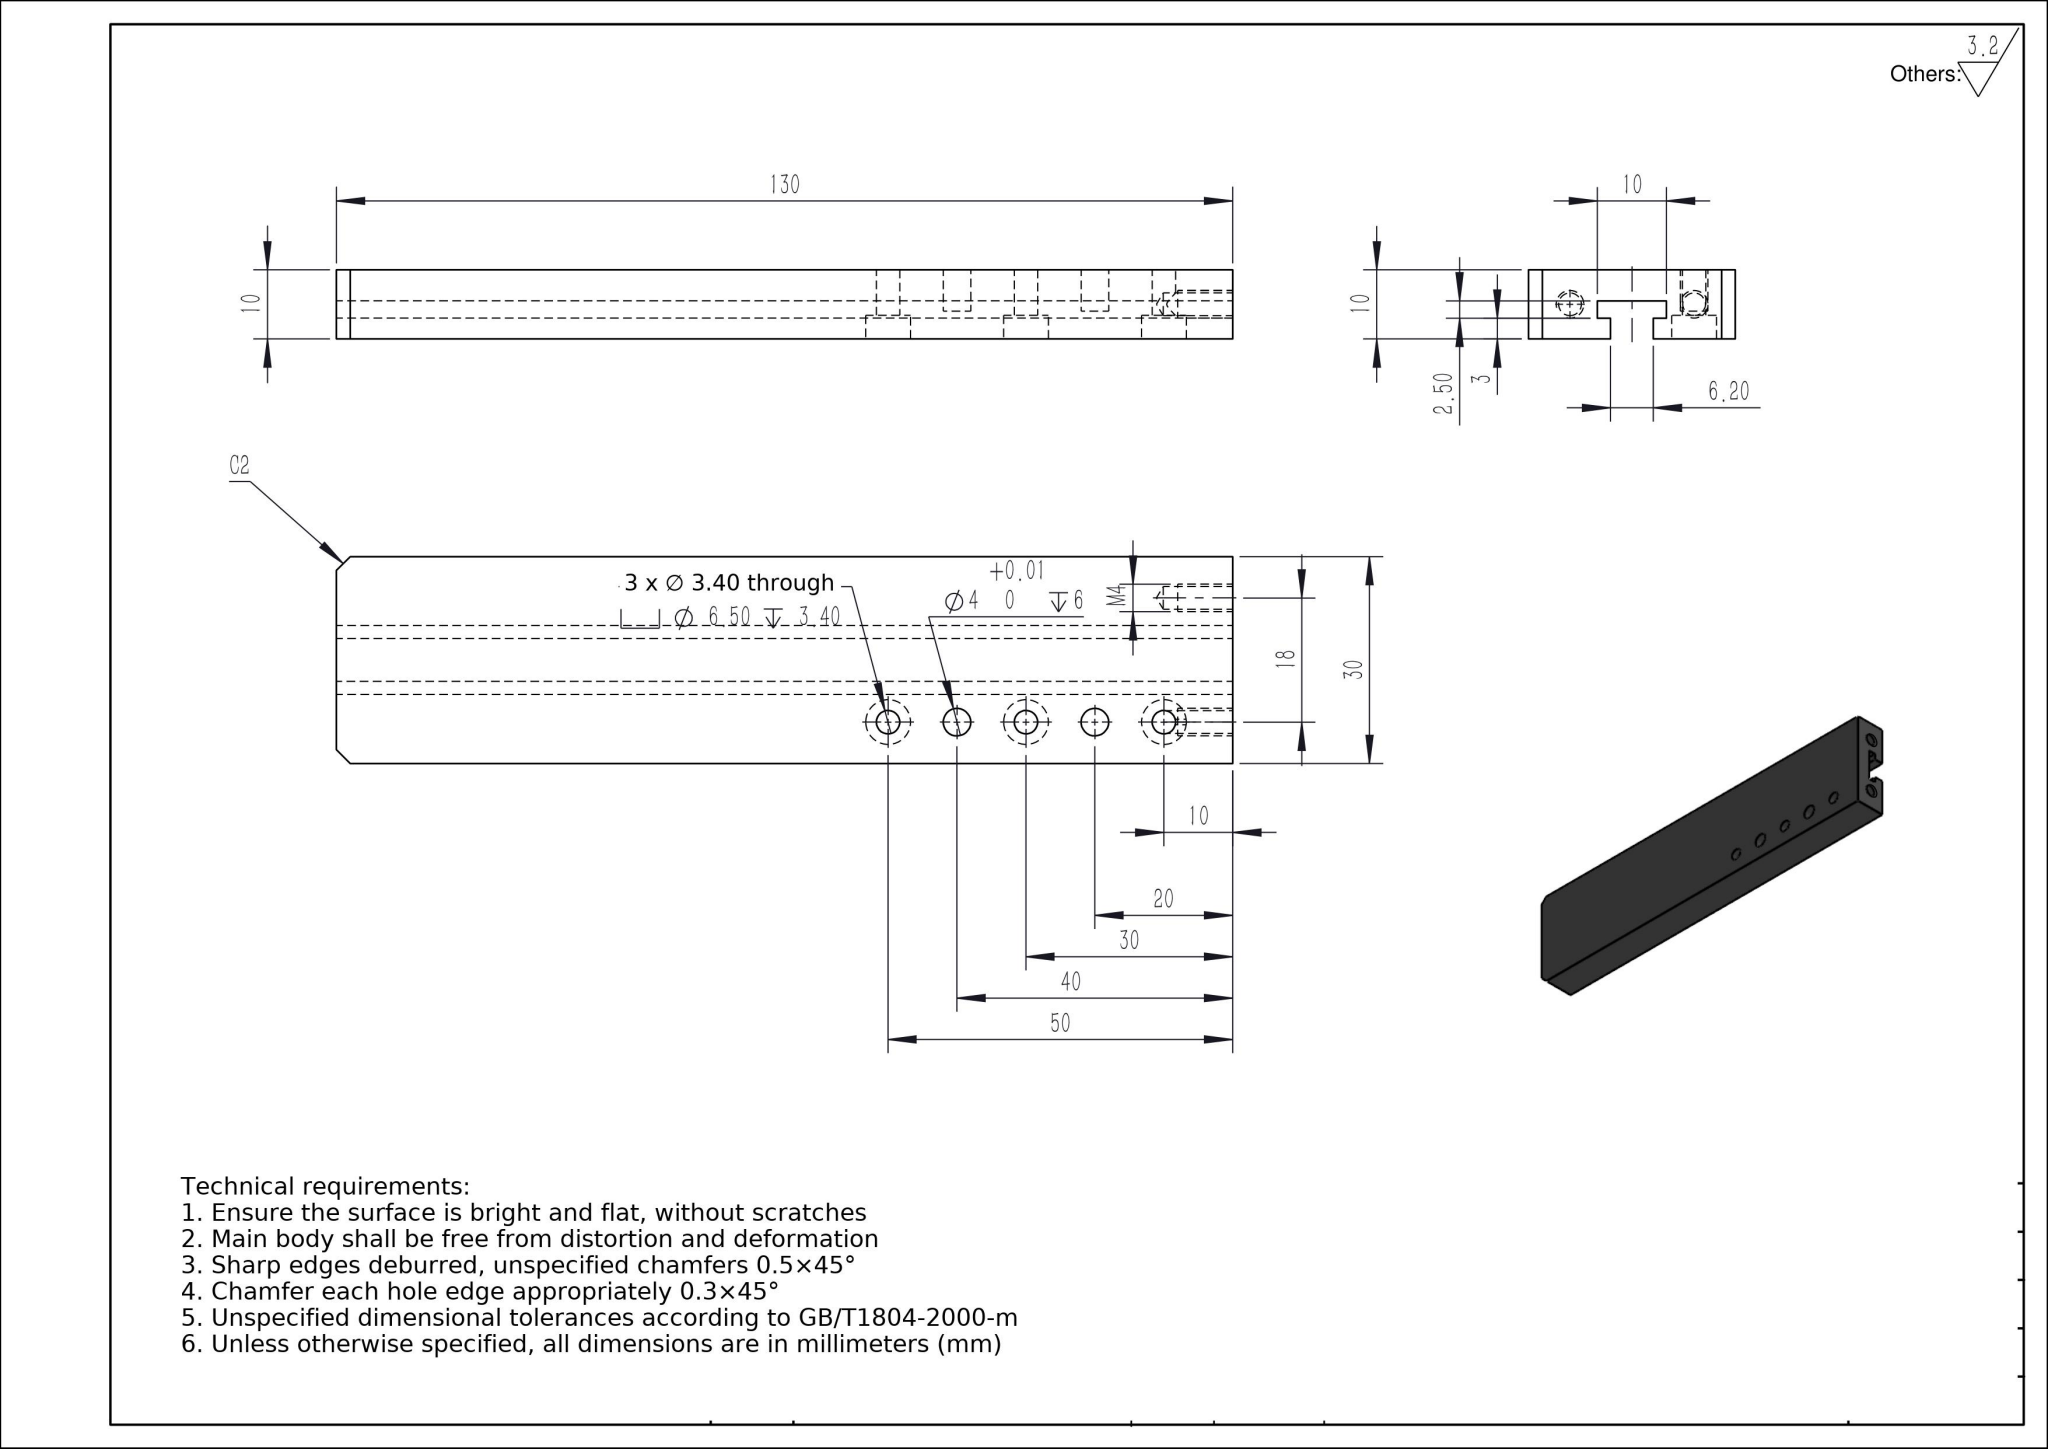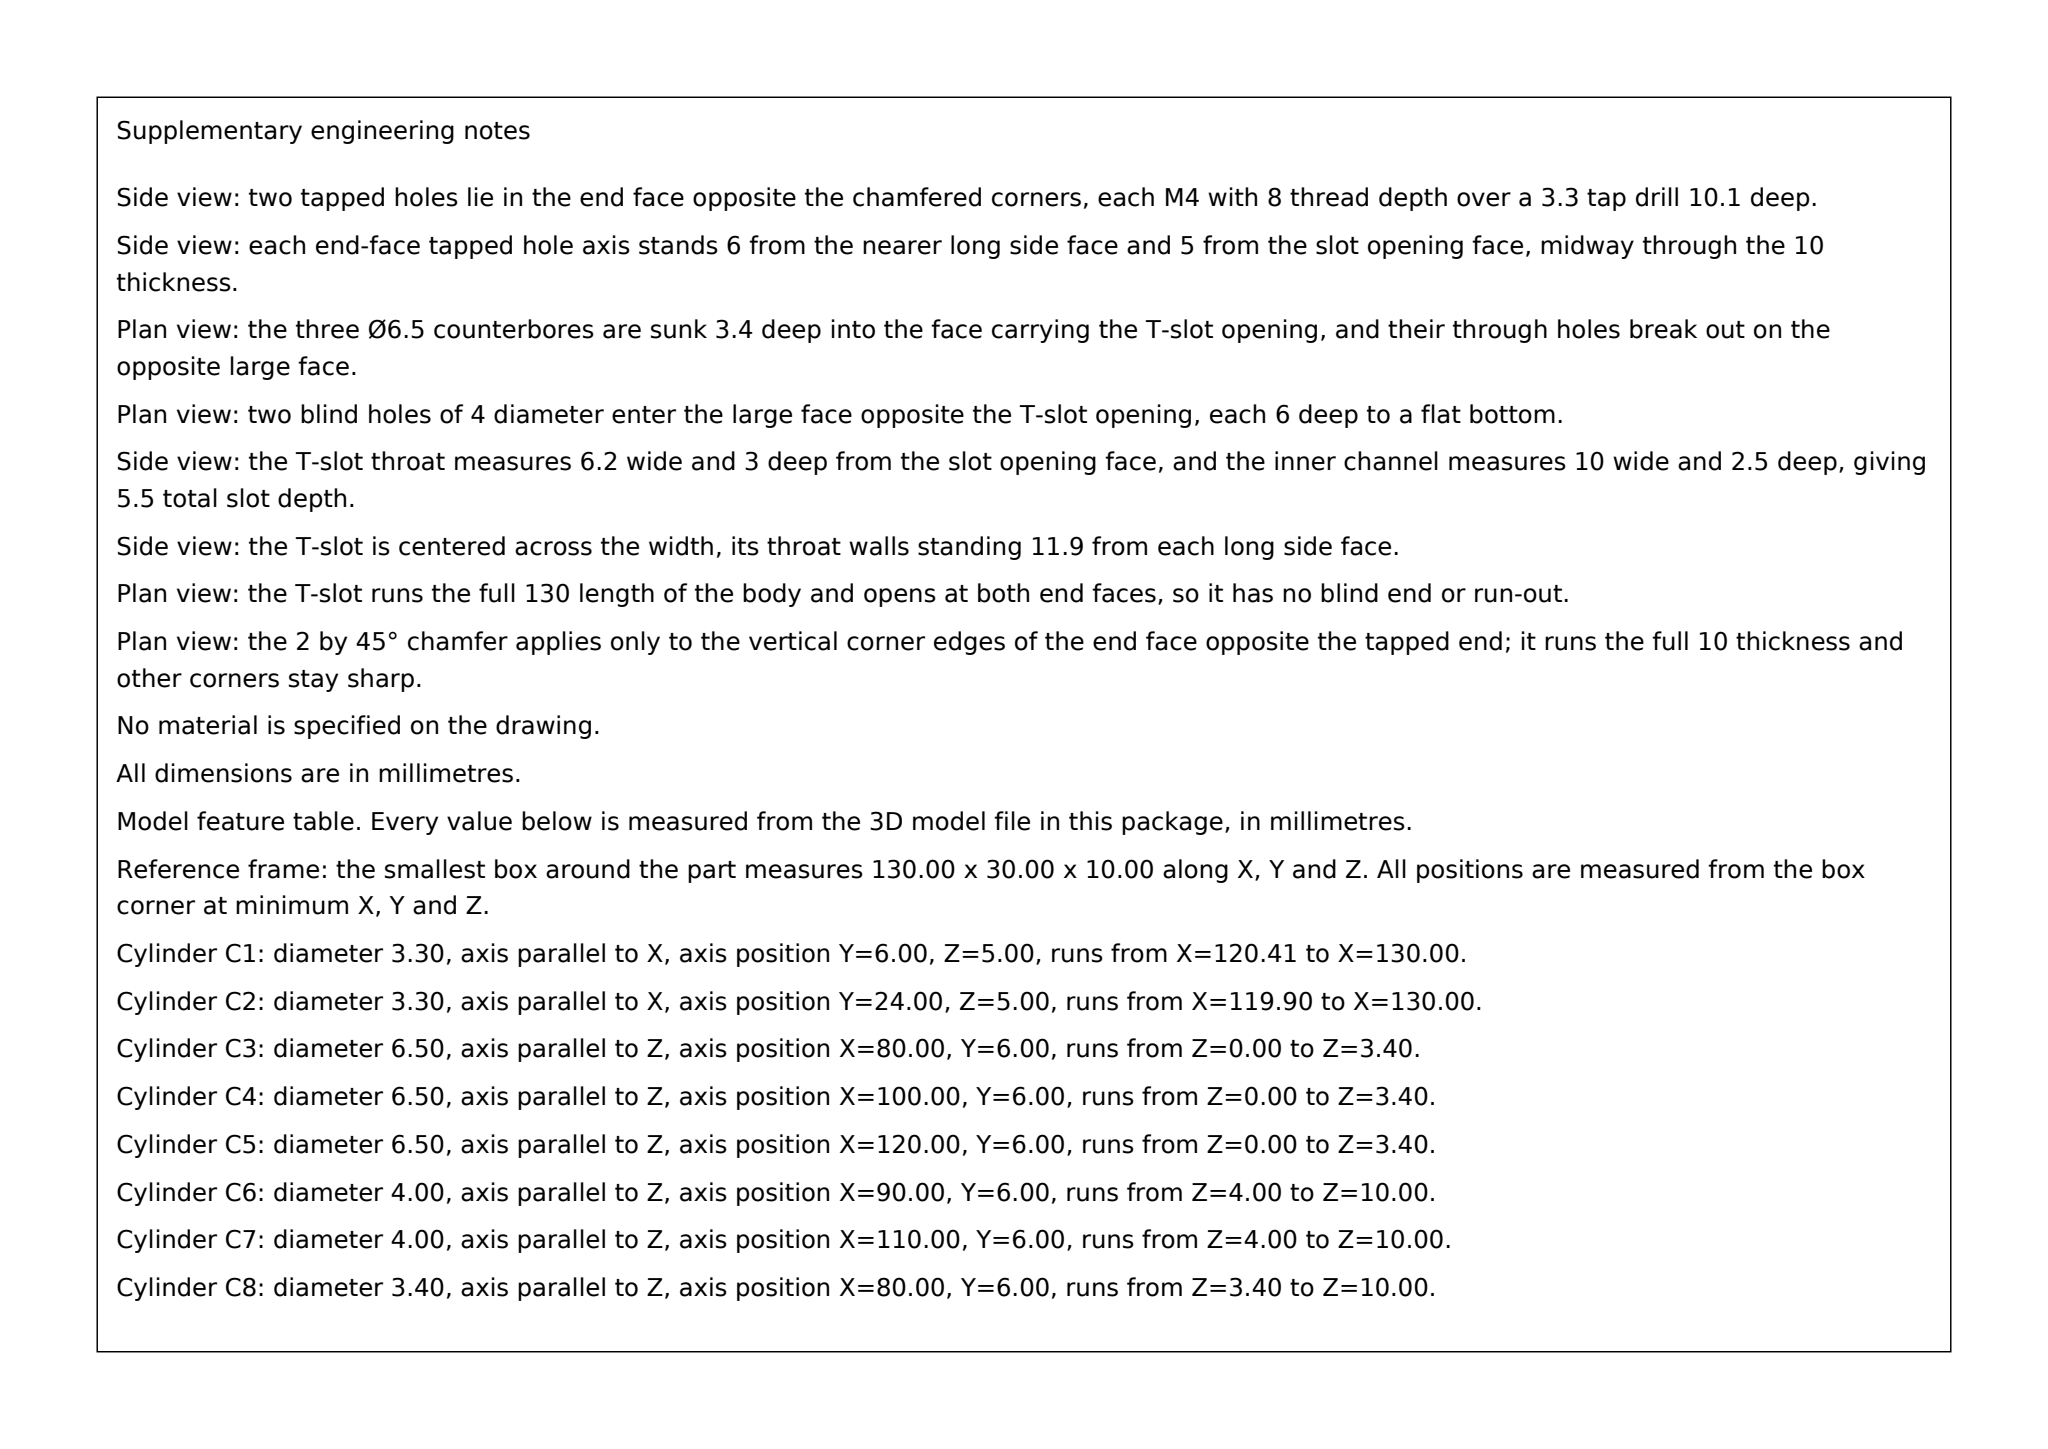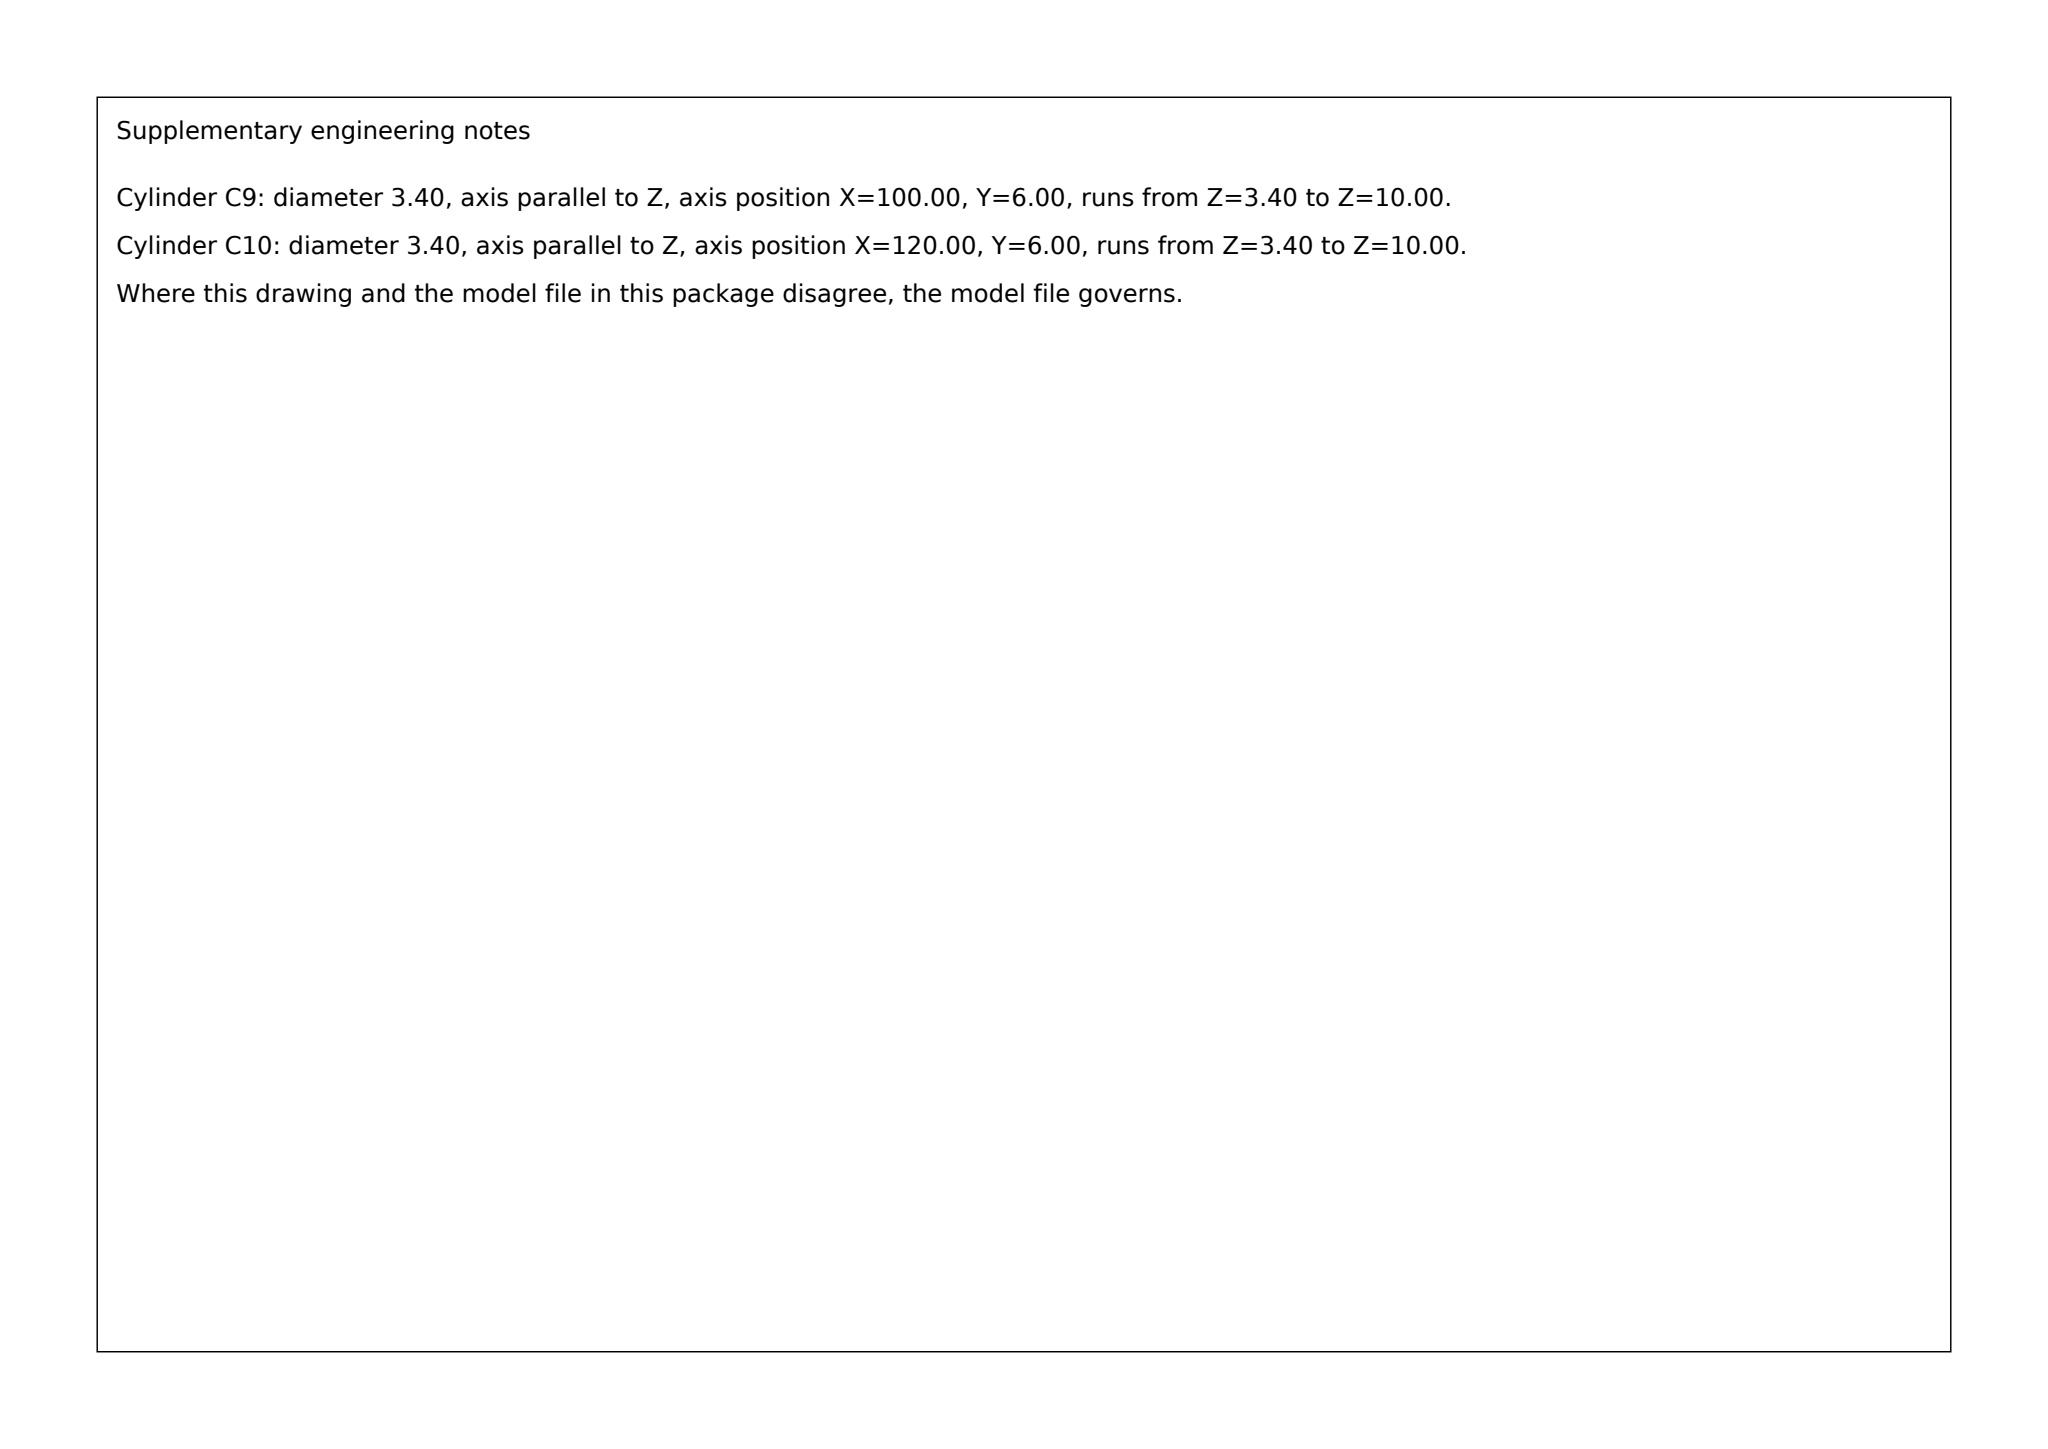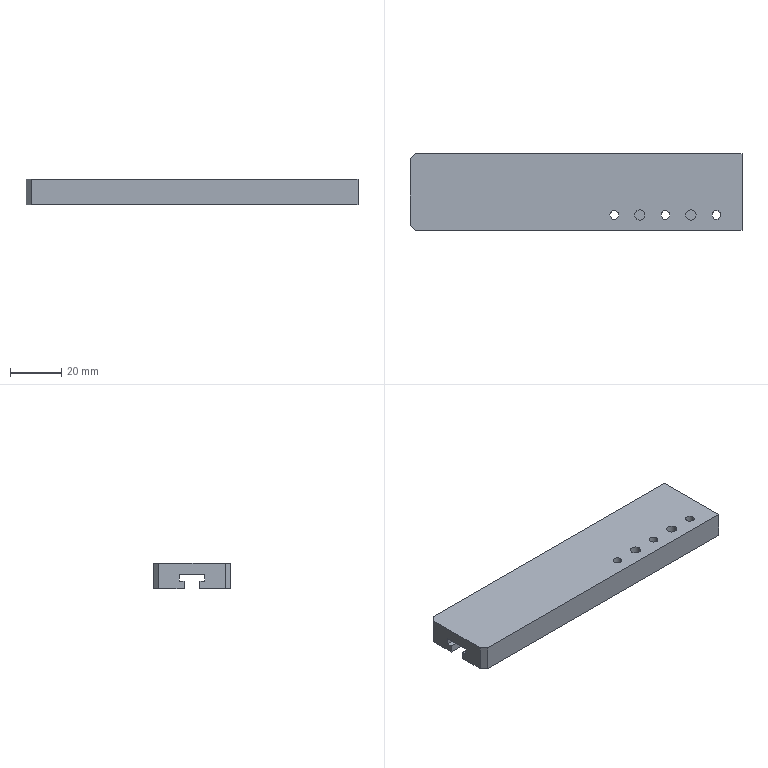Part | SolidWorks | mm | 1 solid | 43 faces | box 130 x 30 x 10 mm | volume 32461 mm3 | plane 21 | cylinder 20 | cone 2 | commonest cylinder face diameters 6.5 x6 3.4 x6 4 x4 3.3 x4
Drawing notes:
2X M4 DP 10 IN RH END FACE AT MID-THK (5 FROM FACE) | from the solid: Ø3.3 x-axis holes y=6 & 24, z=5 = half of 10 thk, depth ~10 from x=130; 118° pt
HOLE ROW CL 6 FROM LOWER LONG EDGE (FRONT VIEW) | from the solid: Ø3.4 & Ø4 holes, z-axis, all at y=6.0; bbox height 30
END VIEW: 2X M4 CL AT 6 & 24 FROM LOWER EDGE | from the solid: Ø3.3 x-axis holes at y=6.0 and y=24.0, from x=130 face
2X Ø4 +0.01/0 DP 6, 20 APART (REPLACES GARBLED NOTE) | from the solid: Ø4 z-holes at x=90 and x=110, y=6, z from 4.0 to 10.0 = 6 deep
build123d program:
from build123d import *

# Parameters (mm, degrees)
SKETCH2_W                                       = 130
SKETCH2_H                                       = 30
BOSS_EXTRUDE1_DEPTH                             = 10
SKETCH3_W                                       = 2.5
SKETCH3_H                                       = 10
CUT_EXTRUDE1_DEPTH                              = 150
SKETCH4_W                                       = 3
SKETCH4_H                                       = 6.2
CUT_EXTRUDE2_DEPTH                              = 150
CHAMFER1_SIZE                                   = 2
M4_TAPPED_HOLE1_D                               = 3.3
M4_TAPPED_HOLE1_DEPTH                           = 10.1
M4_TAPPED_HOLE1_TIP                             = 0.9914
M3_HEX_SOCKET_HEAD_CAP_SCREW_CBORE1_D           = 3.4
M3_HEX_SOCKET_HEAD_CAP_SCREW_CBORE1_CBORE_D     = 6.5
M3_HEX_SOCKET_HEAD_CAP_SCREW_CBORE1_CBORE_DEPTH = 3.4
SKETCH9_R                                       = 2
CUT_EXTRUDE3_DEPTH                              = 6


with BuildPart() as part:
    # Sketch2 → Boss-Extrude1 (new body)
    with BuildSketch(Plane.XY):
        Rectangle(SKETCH2_W, SKETCH2_H)
    extrude(amount=BOSS_EXTRUDE1_DEPTH)

    # Sketch3 → Cut-Extrude1 (cut)
    with BuildSketch(Plane(origin=(65, 0, 0), x_dir=(0, 0, -1), z_dir=(1, 0, 0))):
        with Locations((-4.25, 0)):
            Rectangle(SKETCH3_W, SKETCH3_H)
    extrude(amount=-CUT_EXTRUDE1_DEPTH, mode=Mode.SUBTRACT)

    # Sketch4 → Cut-Extrude2 (cut)
    with BuildSketch(Plane(origin=(65, 0, 0), x_dir=(0, 0, -1), z_dir=(1, 0, 0))):
        with Locations((-1.5, 0)):
            Rectangle(SKETCH4_W, SKETCH4_H)
    extrude(amount=-CUT_EXTRUDE2_DEPTH, mode=Mode.SUBTRACT)

    # Chamfer1
    chamfer1_edges = [part.edges().sort_by_distance(p)[0] for p in [
        (-65, -15, 5),
        (-65, 15, 5),
    ]]
    chamfer(chamfer1_edges, length=CHAMFER1_SIZE)

    # M4 Tapped Hole1
    with Locations(Plane(origin=(65, 0, 0), x_dir=(0, 0, -1), z_dir=(1, 0, 0))):
        with Locations((-5, 9), (-5, -9)):
            Hole(M4_TAPPED_HOLE1_D / 2, depth=M4_TAPPED_HOLE1_DEPTH)
            with Locations((0, 0, -(M4_TAPPED_HOLE1_DEPTH + M4_TAPPED_HOLE1_TIP / 2))):  # 118° drill point
                Cone(0, M4_TAPPED_HOLE1_D / 2, M4_TAPPED_HOLE1_TIP, mode=Mode.SUBTRACT)

    # M3 Hex Socket Head Cap Screw CBORE1 (through all)
    with Locations(Plane(origin=(0, 0, 0), x_dir=(-1, 0, 0), z_dir=(0, 0, -1))):
        with Locations((-55, -9), (-35, -9), (-15, -9)):
            CounterBoreHole(M3_HEX_SOCKET_HEAD_CAP_SCREW_CBORE1_D / 2, M3_HEX_SOCKET_HEAD_CAP_SCREW_CBORE1_CBORE_D / 2, M3_HEX_SOCKET_HEAD_CAP_SCREW_CBORE1_CBORE_DEPTH)

    # Sketch9 → Cut-Extrude3 (cut)
    with BuildSketch(Plane.XY.offset(10)):
        with Locations((45, -9)):
            Circle(SKETCH9_R)
        with Locations((25, -9)):
            Circle(SKETCH9_R)
    extrude(amount=-CUT_EXTRUDE3_DEPTH, mode=Mode.SUBTRACT)


solid = part.part